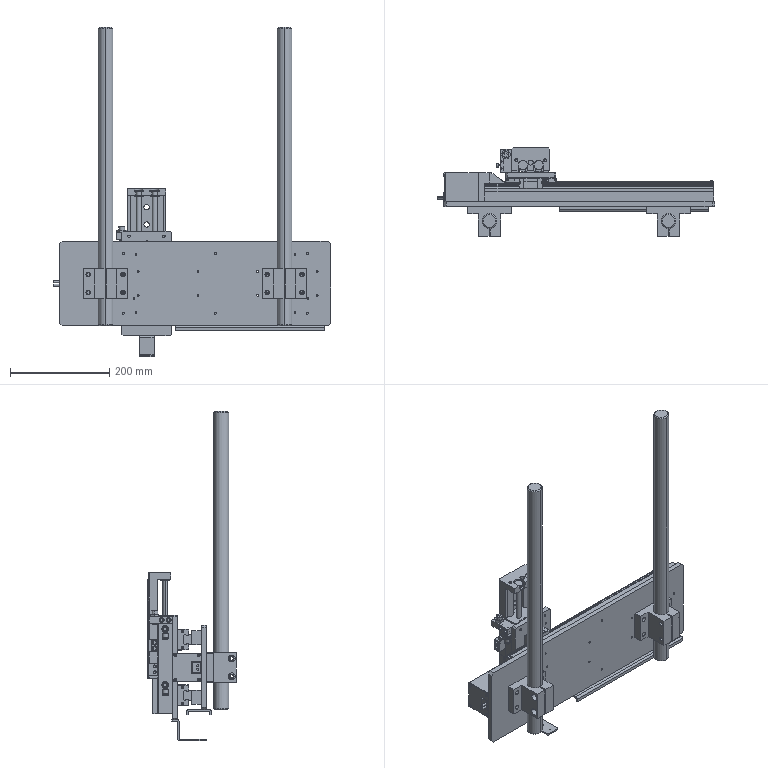Assembly | SolidWorks | mm | 27 component files | 27 solids | 2195 faces | box 557.25 x 178 x 662 mm | volume 5037865 mm3 | plane 1013 | cylinder 878 | cone 228 | spline 46 | torus 24 | sphere 6 | commonest cylinder face diameters 3 x75 4.2 x62 6 x50 10 x48 9.5 x42 3.08 x40 4 x35 4.134 x32
Bill of materials:
OpticalAxisClamp | 2 | 45 | T-shaped block with a large through bore in the central body. A narrow slot runs from the bore to the bottom edge, splitting the body. A wide flange has four through holes, and two cross holes go through the side face of the central body.
SFTJ-02-Column | 2 | 45 | Long, slender solid cylindrical rod with flat ends.
SFTJ-03-XModuleBackPlate | 1 | 45 | Thin rectangular plate with chamfered corners and many small through holes of different sizes, arranged in symmetric clusters.
SFTJ-04-DragChainSheet-Metal | 1 | 201 Annealed Stainless Steel (SS) | Long channel with a U-shaped cross-section and rounded bends, like a formed sheet profile. The web has a few holes.
SFTJ-05-GuidePlate | 2 | 6061 Alloy | Long solid bar with a rectangular cross-section. One long side face has many small holes of mixed sizes along its length.
SFTJ-06-CylinderBackPlate | 1 | 6061 Alloy | Rectangular plate with chamfered corners and a central rectangular cutout with rounded corners. Holes run along the centerline, with a few smaller holes near the corners.
SFTJ-07-DragChainBracket | 1 | 201 Annealed Stainless Steel (SS) | Z-shaped (offset) bent bracket of uniform thickness with rounded bends: a long lower flange, a vertical web, and a short upper flange pointing the opposite way. The upper flange has two larger holes and the lower flange has two smaller holes.
SFTJ-08-ModuleAdapterBlock | 1 |  | Thick rectangular plate with chamfered corners, four larger corner through holes, and two smaller holes on the mid-line.
SMC-AS2201F-01-06S | 2 |  | Elbow-shaped body of revolved features. A main cylindrical body has a hex section, a separate hex nut, a stem ending in a round knob, and a tapered end with a small central bore. A perpendicular cylindrical branch has a circumferential groove and a collar near its end.
0SMC-MXS20-100AS-M9N-1 | 2 |  | Stepped pin. A longer upper section has a keyhole-like cross-section (a circle merged with a rectangular tab), and a smaller-diameter cylindrical shank extends below it. The tab face near the top has a small circular feature with a slot line.
0SMC-MXS20-100AS-M9N-2 | 1 |  | Prismatic extruded profile block with a complex constant cross-section: a raised rectangular rib on top, rounded notches along the top and bottom edges, and two round-ended grooves on one side. A row of evenly spaced holes runs along one long face, and bores show on the end face.
0SMC-MXS20-100AS-M9N-3 | 1 |  | Elongated block with a thick end head. Two parallel rods with end collars run in recessed channels along one face, and a row of evenly spaced holes sits between them. The end face has a central hole, two flanking smaller holes, and two semicircular recesses along one edge.
0SMC-MXS20-100AS-M9N-4 | 1 |  | Rectangular block with a stepped (L-shaped) footprint. A hexagonal prism sits on the top face, and a cylindrical boss with a hexagonal socket sits on top of the prism. A short cylindrical stub sticks out below the block on the same axis.
0SMC-MXS20-100AS-M9N-5 | 1 |  | Plain rectangular box with flat faces and no visible holes, chamfers, or other features.
0MIM-SVR28-460-1 | 2 |  | Elongated block whose end profile is roughly C- or I-shaped. A channel runs along its length on one side, with semicircular, rod-like ridges along the inner edges of the channel. A plate on one end carries two small circular features with cross marks and an angled fitting with a hex base and a tapered head.
0MIM-SVR28-460-2 | 2 |  | Long, straight bar of constant cross-section with a row of eight evenly spaced small circular holes along its length. The cross-section is roughly rectangular, with a semicircular groove on each of two opposite faces and chamfered corners on one side.
Mates:
1. coincident | SFTJ-03-XModuleBackPlate-1 face at (-137.759, -7.279, 38.589) dir (0, 1, 0) | SFTJ-05-GuidePlate-1 face at (-97.009, -7.279, 98.589) dir (0, -1, 0)
2. distance | SFTJ-05-GuidePlate-1 plane at (-97.009, 2.721, 98.589) dir (0, 0, -1) | SFTJ-03-XModuleBackPlate-1 plane at (-137.759, -12.279, 38.589) dir (0, 0, 1)
3. coincident | SFTJ-03-XModuleBackPlate-1 plane at (-137.759, -12.279, 38.589) dir (0, 0, 1) | OpticalAxisHolder-2 plane at (-317.759, -17.279, 38.589) dir (0, 0, -1)
4. coincident | SFTJ-03-XModuleBackPlate-1 face at (-137.759, -17.279, 38.589) dir (0, -1, 0) | OpticalAxisHolder-2/OpticalAxisClamp-2 face at (-362.759, -17.279, 8.589) dir (0, 1, 0)
5. distance | OpticalAxisHolder-2 plane at (-317.759, -17.279, 38.589) dir (1, 0, 0) | SFTJ-03-XModuleBackPlate-1 plane at (-137.759, -12.279, 38.589) dir (1, 0, 0)
6. concentric | OpticalAxisHolder-2/OpticalAxisClamp-2 face at (-317.759, -47.279, 8.589) dir (0, 0, -1) r 15 | SFTJ-02-Column-1 face at (-317.759, -47.279, 553.589) dir (0, 0, -1) r 15
7. coincident | SFTJ-03-XModuleBackPlate-1 face at (-410.259, -17.279, -46.411) dir (0, 0, -1) | SFTJ-02-Column-1 face at (-317.759, -47.279, -46.411) dir (0, 0, -1)
8. parallel | OpticalAxisHolder-2/OpticalAxisClamp-2 face at (-340.259, -77.279, 8.589) dir (-1, 0, 0) | SFTJ-02-Column-1 plane at (-317.759, -47.279, 253.589) dir (1, 0, 0)
9. coincident | SFTJ-03-XModuleBackPlate-1 face at (-137.759, -7.279, 38.589) dir (0, 1, 0) | S25B-300-S3AN3-1/0SMC-LEFS25B-300-S3AN3-2-1 face at (192.606, -7.279, 67.589) dir (0, -1, 0)
10. coincident | SFTJ-03-XModuleBackPlate-1 plane at (-137.759, -12.279, 38.589) dir (1, 0, 0) | S25B-300-S3AN3-1 plane at (-137.759, -7.279, 38.589) dir (-1, 0, 0)
11. distance | SFTJ-03-XModuleBackPlate-1 plane at (-137.759, -12.279, 38.589) dir (0, 0, 1) | S25B-300-S3AN3-1 plane at (-287.009, -7.279, 38.589) dir (0, 0, -1)
12. coincident | SFTJ-06-CylinderBackPlate-1 plane at (-235.009, 45.721, 38.589) dir (1, 0, 0) | S25B-300-S3AN3-1/0SMC-LEFS25B-300-S3AN3-4-1 plane at (-235.009, 36.221, 38.589) dir (1, 0, 0)
13. coincident | SFTJ-06-CylinderBackPlate-1 face at (-235.009, 40.721, 38.589) dir (0, -1, 0) | S25B-300-S3AN3-1/0SMC-LEFS25B-300-S3AN3-4-1 face at (-203.009, 40.721, 63.589) dir (0, 1, 0)
14. coincident | SFTJ-05-GuidePlate-1 face at (-97.009, 12.721, 98.589) dir (0, 1, 0) | SVR28-460-1/0MIM-SVR28-460-2-1 face at (132.991, 12.721, 104.589) dir (0, -1, 0)
15. coincident | SFTJ-05-GuidePlate-1 face at (-327.009, -7.279, 112.589) dir (-1, 0, 0) | SVR28-460-1/0MIM-SVR28-460-2-1 face at (-327.009, 21.401, 84.589) dir (-1, 0, 0)
16. coincident | SFTJ-05-GuidePlate-1 face at (132.991, -7.279, 112.589) dir (1, 0, 0) | S25B-300-S3AN3-1/0SMC-LEFS25B-300-S3AN3-1-1 face at (132.991, 16.621, 67.489) dir (1, 0, 0)
17. coincident | SFTJ-06-CylinderBackPlate-1 plane at (-235.009, 45.721, 38.589) dir (0, 0, 1) | S25B-300-S3AN3-1 plane at (-287.009, -7.279, 38.589) dir (0, 0, -1)
18. coincident | SFTJ-05-GuidePlate-1 face at (132.991, -7.279, 84.589) dir (0, 0, -1) | SVR28-460-1/0MIM-SVR28-460-2-1 face at (132.991, 12.721, 84.589) dir (0, 0, -1)
19. concentric | SFTJ-02-Column-1 face at (-317.759, -47.279, 553.589) dir (0, 0, -1) r 15 | assembly face at (-317.759, -47.279, 518.589) dir (0, 0, -1) r 15
20. coincident | SFTJ-02-Column-1 face at (-317.759, -47.279, 553.589) dir (0, 0, 1) | assembly face at (-347.759, -47.279, 553.589) dir (0, 0, 1)
21. perpendicular | SFTJ-03-XModuleBackPlate-1 face at (-410.259, -17.279, 123.589) dir (-1, 0, 0) | assembly face at (-362.759, -64.279, 517.589) dir (0, -1, 0)
22. coincident | SFTJ-03-XModuleBackPlate-1 face at (-137.759, -7.279, 38.589) dir (0, 1, 0) | SFTJ-05-GuidePlate-4 face at (-97.009, -7.279, -21.411) dir (0, -1, 0)
23. distance | SFTJ-05-GuidePlate-4 plane at (-97.009, 2.721, -21.411) dir (0, 0, 1) | SFTJ-03-XModuleBackPlate-1 plane at (-137.759, -12.279, 38.589) dir (0, 0, 1)
24. coincident | SFTJ-05-GuidePlate-4 face at (132.991, -7.279, -35.411) dir (1, 0, 0) | SFTJ-05-GuidePlate-1 face at (132.991, -7.279, 112.589) dir (1, 0, 0)
25. coincident | SFTJ-05-GuidePlate-4 face at (-97.009, 12.721, -21.411) dir (0, 1, 0) | SVR28-460-4/0MIM-SVR28-460-2-1 face at (132.991, 12.721, -7.411) dir (0, -1, 0)
26. coincident | SFTJ-05-GuidePlate-4 face at (-327.009, -7.279, -7.411) dir (0, 0, 1) | SVR28-460-4/0MIM-SVR28-460-2-1 face at (132.991, 18.901, -7.411) dir (0, 0, 1)
27. coincident | SFTJ-05-GuidePlate-4 face at (-327.009, -7.279, -35.411) dir (-1, 0, 0) | SVR28-460-4/0MIM-SVR28-460-2-1 face at (-327.009, 21.401, -27.411) dir (-1, 0, 0)
28. coincident | SFTJ-03-XModuleBackPlate-1 face at (-410.259, -17.279, -46.411) dir (0, 0, -1) | SFTJ-04-DragChainSheet-Metal-1 face at (-177.009, -27.279, -46.411) dir (0, 0, 1)
29. distance | SFTJ-03-XModuleBackPlate-1 face at (-137.759, -17.279, 38.589) dir (0, -1, 0) | SFTJ-04-DragChainSheet-Metal-1 face at (-177.009, -27.279, -46.411) dir (0, -1, 0)
30. distance | SFTJ-04-DragChainSheet-Metal-1 face at (-177.009, 19.721, -50.148) dir (-1, 0, 0) | SFTJ-05-GuidePlate-4 face at (-327.009, -7.279, -35.411) dir (-1, 0, 0)
31. coincident | SFTJ-06-CylinderBackPlate-1 face at (-235.009, 40.721, 38.589) dir (0, -1, 0) | SFTJ-07-DragChainBracket-1 face at (-250.009, 40.721, -66.411) dir (0, 1, 0)
32. coincident | SFTJ-06-CylinderBackPlate-1 plane at (-235.009, 45.721, 38.589) dir (1, 0, 0) | SFTJ-07-DragChainBracket-1 plane at (-235.009, 37.721, -85.911) dir (-1, 0, 0)
33. coincident | SFTJ-06-CylinderBackPlate-1 face at (-235.009, 50.721, 38.589) dir (0, 1, 0) | SMC-MXS20-100AS-M9N-1/0SMC-MXS20-100AS-M9N-2-1 face at (-273.009, 50.721, 143.589) dir (0, -1, 0)
34. coincident | SFTJ-06-CylinderBackPlate-1 face at (-185.009, 40.721, 143.589) dir (0, 0, 1) | SMC-MXS20-100AS-M9N-1/0SMC-MXS20-100AS-M9N-2-1 face at (-235.009, 50.721, 143.589) dir (0, 0, 1)
35. coincident | SFTJ-06-CylinderBackPlate-1 plane at (-235.009, 45.721, 38.589) dir (1, 0, 0) | SMC-MXS20-100AS-M9N-1 plane at (-235.009, 50.721, -54.911) dir (1, 0, 0)
36. coincident | S25B-300-S3AN3-1 plane at (-287.009, -7.279, 38.589) dir (0, 0, -1) | SFTJ-08-ModuleAdapterBlock-1 plane at (-235.009, 44.721, 38.589) dir (0, 0, -1)
37. coincident | SFTJ-06-CylinderBackPlate-1 face at (-265.009, 40.721, 11.089) dir (1, 0, 0) | SFTJ-08-ModuleAdapterBlock-1 face at (-265.009, 48.721, 12.589) dir (-1, 0, 0)
38. coincident | S25B-300-S3AN3-1/0SMC-LEFS25B-300-S3AN3-4-1 face at (-203.009, 40.721, 63.589) dir (0, 1, 0) | SFTJ-08-ModuleAdapterBlock-1 face at (-235.009, 40.721, 38.589) dir (0, -1, 0)
39. concentric | SMC-MXS20-100AS-M9N-1/0SMC-MXS20-100AS-M9N-2-1 face at (-263.281, 65.721, 3.089) dir (-1, 0, 0) r 4.283 | SMC-AS2201F-01-06S-1 face at (-275.009, 65.721, 3.089) dir (1, 0, 0) r 21.642
40. distance | SMC-MXS20-100AS-M9N-1/0SMC-MXS20-100AS-M9N-2-1 face at (-273.009, 79.721, 143.589) dir (-1, 0, 0) | SMC-AS2201F-01-06S-1 face at (-275.009, 65.721, 3.089) dir (1, 0, 0)
41. distance | SMC-MXS20-100AS-M9N-1/0SMC-MXS20-100AS-M9N-2-1 face at (-273.009, 79.721, 143.589) dir (-1, 0, 0) | SMC-AS2201F-01-06S-2 face at (-275.009, 65.721, 116.089) dir (1, 0, 0)
42. concentric | SMC-MXS20-100AS-M9N-1/0SMC-MXS20-100AS-M9N-2-1 face at (-263.281, 65.721, 116.089) dir (-1, 0, 0) r 4.283 | SMC-AS2201F-01-06S-2 face at (-275.009, 65.721, 116.089) dir (1, 0, 0) r 21.642
43. coincident | 0SMC-LEFS25B-300-S3AN3-2-1 face at (0, 0, 410) dir (0, 0, 1) | 0SMC-LEFS25B-300-S3AN3-1-1 face at (-28.9, 23.9, 410) dir (0, 0, -1)
44. coincident | 0SMC-LEFS25B-300-S3AN3-2-1 plane at (0, 0, 0) dir (1, 0, 0) | 0SMC-LEFS25B-300-S3AN3-1-1 plane at (0, 0.5, 410) dir (1, 0, 0)
45. distance | 0SMC-LEFS25B-300-S3AN3-1-1 plane at (0, 0.5, 410) dir (0, 1, 0) | 0SMC-LEFS25B-300-S3AN3-2-1 plane at (0, 0, 0) dir (0, 1, 0)
46. coincident | 0SMC-LEFS25B-300-S3AN3-2-1 plane at (0, 0, 0) dir (0, 0, 1) | 0SMC-LEFS25B-300-S3AN3-3-1 plane at (0, 0.5, 0) dir (0, 0, 1)
47. coincident | 0SMC-LEFS25B-300-S3AN3-2-1 plane at (0, 0, 0) dir (1, 0, 0) | 0SMC-LEFS25B-300-S3AN3-3-1 plane at (0, 0.5, 0) dir (1, 0, 0)
48. distance | 0SMC-LEFS25B-300-S3AN3-2-1 plane at (0, 0, 0) dir (0, 1, 0) | 0SMC-LEFS25B-300-S3AN3-3-1 plane at (0, 0.5, 0) dir (0, 1, 0)
49. coincident | 0SMC-LEFS25B-300-S3AN3-2-1 face at (-12, 39.5, 411.75) dir (0, 1, 0) | 0SMC-LEFS25B-300-S3AN3-4-1 face at (-12, 39.5, 1) dir (0, -1, 0)
50. coincident | 0SMC-LEFS25B-300-S3AN3-2-1 plane at (0, 0, 0) dir (1, 0, 0) | 0SMC-LEFS25B-300-S3AN3-4-1 plane at (0, 43.5, 52) dir (1, 0, 0)
51. distance | 0SMC-LEFS25B-300-S3AN3-2-1 plane at (0, 0, 0) dir (0, 0, 1) | 0SMC-LEFS25B-300-S3AN3-4-1 plane at (0, 43.5, 52) dir (0, 0, 1)
52. coincident | 0SMC-MXS20-100AS-M9N-2-1 axis at (0, 0, 80.9) dir (0, 0, -1) | 0SMC-MXS20-100AS-M9N-3-1 axis at (0, 0, 19.1) dir (0, 0, 1)
53. coincident | 0SMC-MXS20-100AS-M9N-2-1 axis at (0, 0, 80.9) dir (0, 0, -1) | 0SMC-MXS20-100AS-M9N-3-1 axis at (0, 0, 19.1) dir (0, 0, 1)
54. coincident | 0SMC-MXS20-100AS-M9N-2-1 axis at (0, 0, 80.9) dir (0, 0, -1) | 0SMC-MXS20-100AS-M9N-3-1 axis at (0, 0, 19.1) dir (0, 0, 1)
55. angle | 0SMC-MXS20-100AS-M9N-3-1 plane at (0, 0, 100) dir (1, 0, 0) | 0SMC-MXS20-100AS-M9N-2-1 plane at (0, 0, 0) dir (1, 0, 0)
56. distance | 0SMC-MXS20-100AS-M9N-5-1 plane at (-36, 36, 167.5) dir (-1, 0, 0) | 0SMC-MXS20-100AS-M9N-3-1 plane at (-36, 0, 100) dir (1, 0, 0)
57. coincident | 0SMC-MXS20-100AS-M9N-3-1 axis at (80.9, 36, 173.5) dir (-1, 0, 0) | 0SMC-MXS20-100AS-M9N-5-1 axis at (-116.9, 36, 173.5) dir (1, 0, 0)
58. coincident | 0SMC-MXS20-100AS-M9N-3-1 axis at (80.9, 36, 173.5) dir (-1, 0, 0) | 0SMC-MXS20-100AS-M9N-5-1 axis at (-116.9, 36, 173.5) dir (1, 0, 0)
59. coincident | 0SMC-MXS20-100AS-M9N-3-1 axis at (80.9, 36, 173.5) dir (-1, 0, 0) | 0SMC-MXS20-100AS-M9N-5-1 axis at (-116.9, 36, 173.5) dir (1, 0, 0)
60. angle | 0SMC-MXS20-100AS-M9N-5-1 plane at (-36, 36, 173.5) dir (0, 0, -1) | 0SMC-MXS20-100AS-M9N-3-1 plane at (0, 0, 173.5) dir (0, 0, -1)
61. distance | 0SMC-MXS20-100AS-M9N-4-1 plane at (-36.5, 1, 189) dir (-1, 0, 0) | 0SMC-MXS20-100AS-M9N-2-1 plane at (-36.5, 0, 0) dir (1, 0, 0)
62. coincident | 0SMC-MXS20-100AS-M9N-2-1 axis at (80.9, 8, 189) dir (-1, 0, 0) | 0SMC-MXS20-100AS-M9N-4-1 axis at (-117.4, 8, 189) dir (1, 0, 0)
63. coincident | 0SMC-MXS20-100AS-M9N-2-1 axis at (80.9, 8, 189) dir (-1, 0, 0) | 0SMC-MXS20-100AS-M9N-4-1 axis at (-117.4, 8, 189) dir (1, 0, 0)
64. coincident | 0SMC-MXS20-100AS-M9N-2-1 axis at (80.9, 8, 189) dir (-1, 0, 0) | 0SMC-MXS20-100AS-M9N-4-1 axis at (-117.4, 8, 189) dir (1, 0, 0)
65. angle | 0SMC-MXS20-100AS-M9N-4-1 plane at (-36.5, 1, 189) dir (0, 0, -1) | 0SMC-MXS20-100AS-M9N-2-1 plane at (0, 0, 189) dir (0, 0, -1)
66. coincident | 0SMC-MXS20-100AS-M9N-2-1 axis at (30.3, 18, 80.9) dir (0, 0, -1) | 0SMC-MXS20-100AS-M9N-1-1 axis at (30.3, 18, 94.7) dir (0, 0, 1)
67. coincident | 0SMC-MXS20-100AS-M9N-2-1 axis at (30.3, 18, 80.9) dir (0, 0, -1) | 0SMC-MXS20-100AS-M9N-1-1 axis at (30.3, 18, 94.7) dir (0, 0, 1)
68. angle | 0SMC-MXS20-100AS-M9N-1-1 plane at (30.3, 18, 175.6) dir (0, -1, 0) | 0SMC-MXS20-100AS-M9N-2-1 plane at (30.3, 0, 0) dir (1, 0, 0)
69. coincident | 0SMC-MXS20-100AS-M9N-2-1 axis at (30.3, 12, -80.9) dir (0, 0, 1) | 0SMC-MXS20-100AS-M9N-1-2 axis at (30.3, 12, 156.5) dir (0, 0, -1)
70. coincident | 0SMC-MXS20-100AS-M9N-2-1 axis at (30.3, 12, -80.9) dir (0, 0, 1) | 0SMC-MXS20-100AS-M9N-1-2 axis at (30.3, 12, 156.5) dir (0, 0, -1)
71. angle | 0SMC-MXS20-100AS-M9N-1-2 plane at (30.3, 12, 75.6) dir (0, -1, 0) | 0SMC-MXS20-100AS-M9N-2-1 plane at (30.3, 0, 0) dir (1, 0, 0)
72. distance | 0SMC-MXS20-100AS-M9N-3-1 face at (0, 0, 314) dir (0, 0, 1) | 0SMC-MXS20-100AS-M9N-2-1 face at (0, 0, 0) dir (0, 0, -1)
73. coincident | 0MIM-SVR28-460-2-1 axis at (0, 15.5, 80.9) dir (0, 0, -1) | 0MIM-SVR28-460-1-1 axis at (0, 15.5, -57.1) dir (0, 0, -1)
74. coincident | 0MIM-SVR28-460-2-1 axis at (0, 15.5, 80.9) dir (0, 0, -1) | 0MIM-SVR28-460-1-1 axis at (0, 15.5, -57.1) dir (0, 0, -1)
75. coincident | 0MIM-SVR28-460-2-1 axis at (0, 15.5, 80.9) dir (0, 0, -1) | 0MIM-SVR28-460-1-1 axis at (0, 15.5, -57.1) dir (0, 0, -1)
76. angle | 0MIM-SVR28-460-1-1 plane at (0, 5.5, -138) dir (1, 0, 0) | 0MIM-SVR28-460-2-1 plane at (0, 0, 0) dir (1, 0, 0)
77. distance | 0MIM-SVR28-460-1-1 face at (-10, 8.68, -161.5) dir (0, 0, -1) | 0MIM-SVR28-460-2-1 face at (10, 8.68, -230) dir (0, 0, -1)